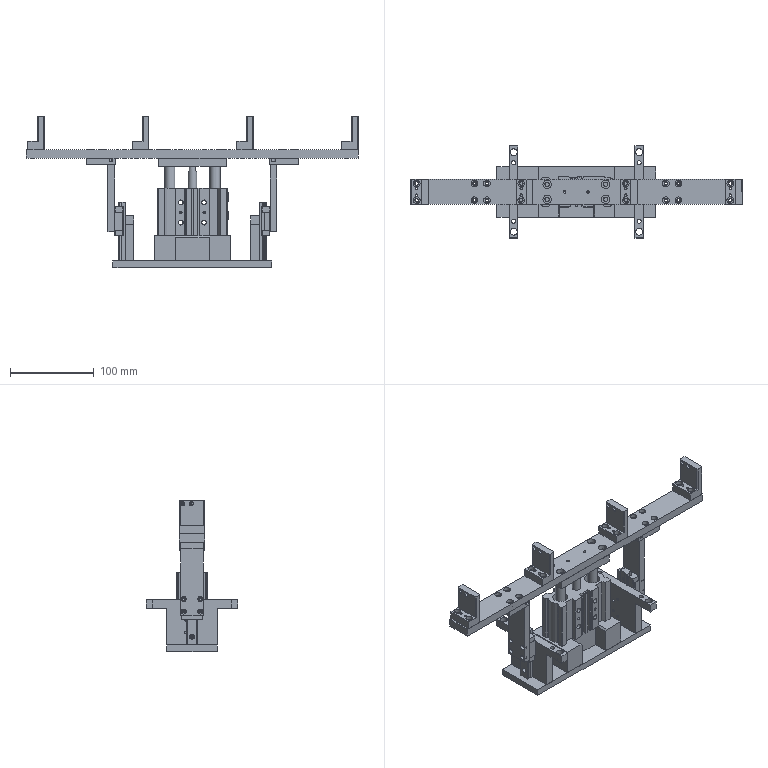Assembly | SolidWorks | mm | 21 component files | 21 solids | 1058 faces | box 397 x 110 x 181 mm | volume 674023 mm3 | cylinder 547 | plane 437 | cone 72 | spline 2 | commonest cylinder face diameters 3 x80 5 x48 4.5 x44 2 x44 6 x44 8 x38 3.3 x24 2.5 x20
Bill of materials:
1-VASP2004MANIFOLD_SOLID_BREP_100 | 2 |  | Rectangular block with a stepped outline. A wide central body sits between narrower end sections. One face has an open channel with rounded corner reliefs, and four holes run through the mounting face.
1-VASP2004MANIFOLD_SOLID_BREP_99-01 | 2 |  | Long straight bar of constant rectangular cross-section. It has a lengthwise groove along each side and three evenly spaced through-holes along its length.
1-VASP2004STG-Body_A_default | 1 |  | Extruded block with a complex profile. Two large round bores run its full length, with a smaller central bore between them. The outer faces carry lengthwise T-slot-like grooves, the side faces have hole patterns, and two hex-socket plugs or screws protrude from one end face.
1-VASP2004STG-SW-T_H_default | 2 |  | Square or rectangular prism with a small notch or step at the top. A short cylindrical collar and a longer, smaller cylindrical shaft extend coaxially from its lower end.
1-VASP2004STG-M-PlateGuideRod_default | 1 |  | Flat rectangular plate with two parallel cylindrical rods and a central stepped rod hanging from one face. A cylindrical collar or bushing sits near the free end of the central rod. The plate has corner holes, two small holes and recessed fastener heads.
JQ-2-0-001 | 1 |  | Thin flat rectangular plate with a symmetric hole pattern: four corner holes and two triangular groups of three smaller holes in the middle.
JQ-2-0-002 | 2 |  | T-shaped plate in profile: a long narrow top bar with a wider plate hanging from its center. The top bar has two larger and two smaller vertical holes, and the hanging plate has four small holes in a staggered pattern.
JQ-2-0-003 | 1 |  | Long, thin, flat rectangular bar with many holes along its length. These include groups of four larger holes, rows of small holes near each end and at intermediate positions, and a few very small center holes.
JQ-2-0-004 | 2 |  | Rectangular block shaped like a thick plate. It has two holes on the narrow top face and four holes in a rectangular pattern on the lower part of the large face.
JQ-2-0-005 | 2 |  | Thick rectangular plate with six through-holes: two larger and four medium-sized. One larger hole near a corner has a side slot opening through the adjacent edge, and the counterbore is partly cut by the plate edge.
JQ-2-0-006 | 1 |  | Rectangular block with an open rectangular notch cut through its thickness from one long edge. The notch edges are chamfered, and four holes sit near the corners of the top face.
JQ-2-0-007 | 4 |  | L-shaped bracket with a tall vertical plate and a short horizontal foot. The foot has holes through it, the vertical plate has two small holes near its top, and the edges are chamfered.
Mates:
1. coincident | JQ-2-0-001-1 face at (-357.058, 59.339, -15.869) dir (0, 0, 1) | JQ-2-0-002-1 face at (-332.058, -0.6609, -15.869) dir (0, 0, -1)
2. concentric | JQ-2-0-001-1 face at (-337.058, 54.339, -15.869) dir (0, 0, -1) r 3.2 | JQ-2-0-002-1 face at (-337.058, 54.339, -15.869) dir (0, 0, -1) r 2.5
3. concentric | JQ-2-0-001-1 face at (-337.058, 4.339, -15.869) dir (0, 0, -1) r 3.2 | JQ-2-0-002-1 face at (-337.058, 4.339, -15.869) dir (0, 0, -1) r 2.5
4. coincident | JQ-2-0-003-1 face at (-461.058, 44.339, 117.131) dir (0, 0, 1) | JQ-2-0-007-1 face at (-459.058, 44.339, 117.131) dir (0, 0, -1)
5. concentric | JQ-2-0-003-1 face at (-453.058, 19.339, 117.131) dir (0, 0, 1) r 2 | JQ-2-0-007-1 face at (-453.058, 19.339, 127.131) dir (0, 0, 1) r 2.25
6. concentric | JQ-2-0-003-1 face at (-453.058, 39.339, 117.131) dir (0, 0, 1) r 2 | JQ-2-0-007-1 face at (-453.058, 39.339, 127.131) dir (0, 0, 1) r 2.25
7. concentric | 1-VASP2004MANIFOLD_SOLID_BREP_99-01-2 face at (-176.558, 23.339, 54.131) dir (0, 0, -1) r 1.25 | 1-VASP2004MANIFOLD_SOLID_BREP_100-1 face at (-176.558, 23.339, 66.631) dir (0, 0, -1) r 1.25
8. concentric | 1-VASP2004MANIFOLD_SOLID_BREP_99-01-2 face at (-176.558, 35.339, 54.131) dir (0, 0, -1) r 1.25 | 1-VASP2004MANIFOLD_SOLID_BREP_100-1 face at (-176.558, 35.339, 66.631) dir (0, 0, -1) r 1.25
9. coincident | JQ-2-0-002-6 face at (-182.058, -0.6609, 38.131) dir (1, 0, 0) | 1-VASP2004MANIFOLD_SOLID_BREP_99-01-2 face at (-182.058, 35.339, 54.131) dir (-1, 0, 0)
10. concentric | JQ-2-0-002-6 face at (-182.058, 29.339, -5.869) dir (1, 0, 0) r 1.25 | 1-VASP2004MANIFOLD_SOLID_BREP_99-01-2 face at (-174.058, 29.339, -5.869) dir (-1, 0, 0) r 3
11. concentric | JQ-2-0-002-6 face at (-182.058, 29.339, 19.131) dir (1, 0, 0) r 1.25 | 1-VASP2004MANIFOLD_SOLID_BREP_99-01-2 face at (-174.058, 29.339, 19.131) dir (-1, 0, 0) r 3
12. concentric | 1-VASP2004MANIFOLD_SOLID_BREP_99-01-3 face at (-347.558, 35.339, 54.131) dir (0, 0, -1) r 1.25 | 1-VASP2004MANIFOLD_SOLID_BREP_100-2 face at (-347.558, 35.339, 66.631) dir (0, 0, -1) r 1.25
13. concentric | 1-VASP2004MANIFOLD_SOLID_BREP_99-01-3 face at (-347.558, 23.339, 54.131) dir (0, 0, -1) r 1.25 | 1-VASP2004MANIFOLD_SOLID_BREP_100-2 face at (-347.558, 23.339, 66.631) dir (0, 0, -1) r 1.25
14. coincident | JQ-2-0-002-1 face at (-342.058, -0.6609, 38.131) dir (-1, 0, 0) | 1-VASP2004MANIFOLD_SOLID_BREP_99-01-3 face at (-342.058, 23.339, 54.131) dir (1, 0, 0)
15. concentric | JQ-2-0-002-1 face at (-332.058, 29.339, 19.131) dir (1, 0, 0) r 1.25 | 1-VASP2004MANIFOLD_SOLID_BREP_99-01-3 face at (-333.081, 29.339, 19.131) dir (1, 0, 0) r 1.75
16. concentric | JQ-2-0-002-1 face at (-332.058, 29.339, -5.869) dir (1, 0, 0) r 1.25 | 1-VASP2004MANIFOLD_SOLID_BREP_99-01-3 face at (-333.081, 29.339, -5.869) dir (1, 0, 0) r 1.75
17. coincident | 1-VASP2004MANIFOLD_SOLID_BREP_100-1 face at (-169.058, 42.839, 48.981) dir (1, 0, 0) | JQ-2-0-004-1 face at (-169.058, 15.839, 99.131) dir (-1, 0, 0)
18. concentric | 1-VASP2004MANIFOLD_SOLID_BREP_100-1 edge at (-172.558, 19.339, 39.131) dir (1, 0, 0) r 1.5 | JQ-2-0-004-1 face at (-161.058, 19.339, 39.131) dir (1, 0, 0) r 1.7
19. concentric | 1-VASP2004MANIFOLD_SOLID_BREP_100-1 face at (-169.058, 39.339, 24.131) dir (-1, 0, 0) r 1.5 | JQ-2-0-004-1 face at (-161.058, 39.339, 24.131) dir (1, 0, 0) r 1.7
20. coincident | JQ-2-0-004-1 face at (-161.058, 15.839, 99.131) dir (0, 0, 1) | JQ-2-0-005-1 face at (-135.058, 42.839, 99.131) dir (0, 0, -1)
21. concentric | JQ-2-0-004-1 face at (-165.058, 19.339, 99.131) dir (0, 0, 1) r 1.65 | JQ-2-0-005-1 face at (-165.058, 19.339, 107.131) dir (0, 0, 1) r 4
22. concentric | JQ-2-0-004-1 face at (-165.058, 39.339, 99.131) dir (0, 0, 1) r 1.65 | JQ-2-0-005-1 face at (-165.058, 39.339, 107.131) dir (0, 0, 1) r 2.25
23. coincident | JQ-2-0-003-1 face at (-461.058, 44.339, 107.131) dir (0, 0, -1) | JQ-2-0-005-1 face at (-135.058, 42.839, 107.131) dir (0, 0, 1)
24. coincident | 1-VASP2004MANIFOLD_SOLID_BREP_100-2 face at (-355.058, 15.839, 48.981) dir (-1, 0, 0) | JQ-2-0-004-2 face at (-355.058, 42.839, 99.131) dir (1, 0, 0)
25. concentric | 1-VASP2004MANIFOLD_SOLID_BREP_100-2 face at (-355.058, 39.339, 24.131) dir (1, 0, 0) r 1.5 | JQ-2-0-004-2 face at (-363.058, 39.339, 24.131) dir (-1, 0, 0) r 1.7
26. concentric | 1-VASP2004MANIFOLD_SOLID_BREP_100-2 face at (-355.058, 19.339, 39.131) dir (1, 0, 0) r 1.5 | JQ-2-0-004-2 face at (-363.058, 19.339, 39.131) dir (-1, 0, 0) r 1.7
27. coincident | JQ-2-0-004-2 face at (-363.058, 42.839, 99.131) dir (0, 0, 1) | JQ-2-0-005-2 face at (-389.058, 15.839, 99.131) dir (0, 0, -1)
28. concentric | JQ-2-0-004-2 face at (-359.058, 39.339, 99.131) dir (0, 0, 1) r 1.65 | JQ-2-0-005-2 face at (-359.058, 39.339, 107.131) dir (0, 0, 1) r 4
29. concentric | JQ-2-0-004-2 face at (-359.058, 19.339, 99.131) dir (0, 0, 1) r 1.65 | JQ-2-0-005-2 face at (-359.058, 19.339, 107.131) dir (0, 0, 1) r 4
30. coincident | JQ-2-0-003-1 face at (-461.058, 44.339, 107.131) dir (0, 0, -1) | JQ-2-0-005-2 face at (-389.058, 15.839, 107.131) dir (0, 0, 1)
31. coincident | JQ-2-0-001-1 face at (-357.058, 59.339, -15.869) dir (0, 0, 1) | JQ-2-0-006-1 face at (-307.058, 59.339, -15.869) dir (0, 0, -1)
32. concentric | JQ-2-0-001-1 face at (-226.058, 41.339, -23.869) dir (0, 0, 1) r 2.7 | JQ-2-0-006-1 face at (-226.058, 41.339, 44.131) dir (0, 0, -1) r 3
33. concentric | JQ-2-0-001-1 face at (-298.058, 17.339, -23.869) dir (0, 0, 1) r 2.7 | JQ-2-0-006-1 face at (-298.058, 17.339, 44.131) dir (0, 0, -1) r 3
34. concentric | 1-VASP2004STG-M-20-20-T0H-D-1/1-VASP2004STG-Body_A_default-1 face at (-289.058, 29.339, 14.131) dir (0, 0, 1) r 9.1 | 1-VASP2004STG-M-PlateGuideRod_default-1 face at (-289.058, 29.339, 21.16) dir (0, 0, 1) r 6
35. concentric | 1-VASP2004STG-M-20-20-T0H-D-1/1-VASP2004STG-Body_A_default-1 face at (-235.058, 29.339, 14.131) dir (0, 0, 1) r 9.1 | 1-VASP2004STG-M-PlateGuideRod_default-1 face at (-235.058, 29.339, 21.16) dir (0, 0, 1) r 6
36. distance | 1-VASP2004STG-M-20-20-T0H-D-1/1-VASP2004STG-Body_A_default-1 face at (-303.558, 47.339, 71.131) dir (0, 0, 1) | 1-VASP2004STG-M-PlateGuideRod_default-1 face at (-221.558, 44.339, 97.131) dir (0, 0, -1)
37. coincident | JQ-2-0-006-1 face at (-307.058, 59.339, 14.131) dir (0, 0, 1) | 1-VASP2004STG-M-20-20-T0H-D-1/1-VASP2004STG-Body_A_default-1 face at (-262.058, 29.339, 14.131) dir (0, 0, -1)
38. concentric | JQ-2-0-001-1 face at (-226.058, 41.339, -23.869) dir (0, 0, 1) r 2.7 | 1-VASP2004STG-M-20-20-T0H-D-1/1-VASP2004STG-Body_A_default-1 face at (-226.058, 41.339, 14.131) dir (0, 0, -1) r 2.5
39. concentric | JQ-2-0-006-1 face at (-298.058, 17.339, 44.131) dir (0, 0, -1) r 3 | 1-VASP2004STG-M-20-20-T0H-D-1/1-VASP2004STG-Body_A_default-1 face at (-298.058, 17.339, 14.131) dir (0, 0, -1) r 2.5
40. coincident | JQ-2-0-003-1 face at (-461.058, 44.339, 107.131) dir (0, 0, -1) | 1-VASP2004STG-M-PlateGuideRod_default-1 face at (-221.558, 44.339, 107.131) dir (0, 0, 1)
41. concentric | JQ-2-0-003-1 face at (-227.058, 20.339, 117.131) dir (0, 0, 1) r 2.75 | 1-VASP2004STG-M-PlateGuideRod_default-1 face at (-227.058, 20.339, 107.131) dir (0, 0, 1) r 2.5
42. concentric | JQ-2-0-003-1 face at (-297.058, 38.339, 117.131) dir (0, 0, 1) r 2.75 | 1-VASP2004STG-M-PlateGuideRod_default-1 face at (-297.058, 38.339, 107.131) dir (0, 0, 1) r 2.5